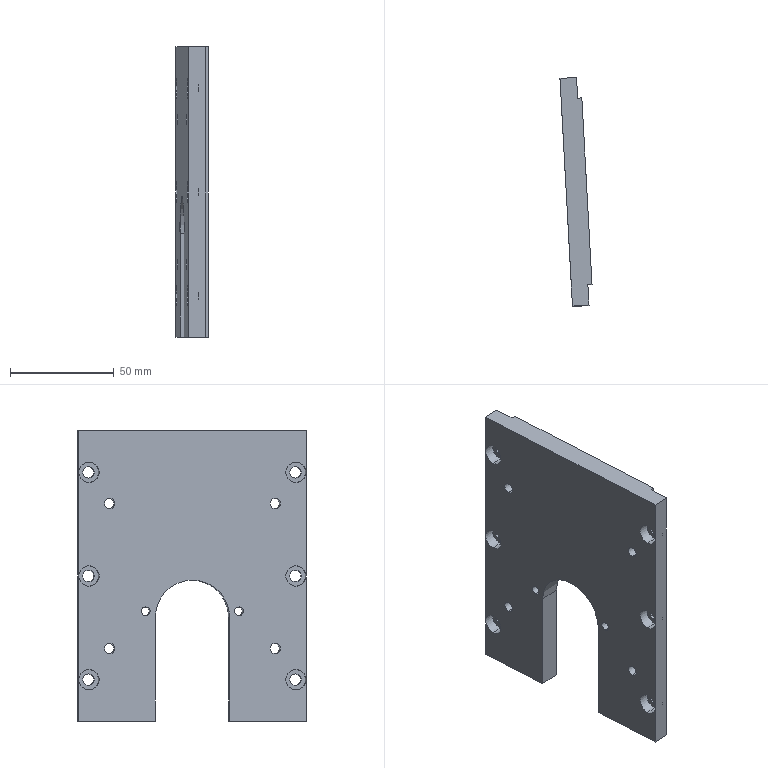Component | SolidWorks | BearingPressPartG-1 | 1 solid | 56 faces | box 15.46 x 110.27 x 140 mm | volume 121558 mm3 | cylinder 37 | plane 19 | commonest cylinder face diameters 9.8 x12 5.5 x12 5 x8 4.2 x4 36 x1
build123d program:
from build123d import *

# Parameters (mm, degrees)
BOSS_EXTRUDE1_DEPTH                             = 140
M5_HEX_SOCKET_HEAD_CAP_SCREW_CBORE1_D           = 5.5
M5_HEX_SOCKET_HEAD_CAP_SCREW_CBORE1_CBORE_D     = 9.8
M5_HEX_SOCKET_HEAD_CAP_SCREW_CBORE1_CBORE_DEPTH = 5
CUT_EXTRUDE1_DEPTH                              = 179.326
M6_TAPPED_HOLE1_D                               = 5
M6_TAPPED_HOLE1_DEPTH                           = 36.5
M6_TAPPED_HOLE1_TIP                             = 1.502
M5_TAPPED_HOLE1_D                               = 4.2


with BuildPart() as part:
    # Sketch1 → Boss-Extrude1 (new body)
    with BuildSketch(Plane.XY):
        Polygon((0, 0), (8, 0), (8, -10), (10, -10), (10, -100), (8, -100), (8, -110), (0, -110), align=None)
    extrude(amount=BOSS_EXTRUDE1_DEPTH)

    # M5 Hex Socket Head Cap Screw CBORE1 (through all)
    with Locations(Plane.ZY):
        with Locations((70, -5), (120, -5), (20, -5), (20, -105), (70, -105), (120, -105)):
            CounterBoreHole(M5_HEX_SOCKET_HEAD_CAP_SCREW_CBORE1_D / 2, M5_HEX_SOCKET_HEAD_CAP_SCREW_CBORE1_CBORE_D / 2, M5_HEX_SOCKET_HEAD_CAP_SCREW_CBORE1_CBORE_DEPTH)

    # Sketch6 → Cut-Extrude1 (cut, through all)
    with BuildSketch(Plane.ZY):
        with BuildLine():
            Line((90, -37), (195.17, -37))
            Line((195.17, -37), (195.17, -73))
            Line((195.17, -73), (90, -73))
            ThreePointArc((90, -73), (72, -55), (90, -37))
        make_face()
    extrude(amount=-CUT_EXTRUDE1_DEPTH, mode=Mode.SUBTRACT)

    # M6 Tapped Hole1
    with Locations(Plane.ZY):
        with Locations((35, -15), (105, -15), (105, -95), (35, -95)):
            Hole(M6_TAPPED_HOLE1_D / 2, depth=M6_TAPPED_HOLE1_DEPTH)
            with Locations((0, 0, -(M6_TAPPED_HOLE1_DEPTH + M6_TAPPED_HOLE1_TIP / 2))):  # 118° drill point
                Cone(0, M6_TAPPED_HOLE1_D / 2, M6_TAPPED_HOLE1_TIP, mode=Mode.SUBTRACT)

    # M5 Tapped Hole1 (through all)
    with Locations(Plane.ZY):
        with Locations((87, -32.5), (87, -77.5)):
            Hole(M5_TAPPED_HOLE1_D / 2)


solid = part.part

# Placed as in the assembly
solid = solid.moved(Location((388.553, 64.634, -143.818), (180, 0, -3.137)))